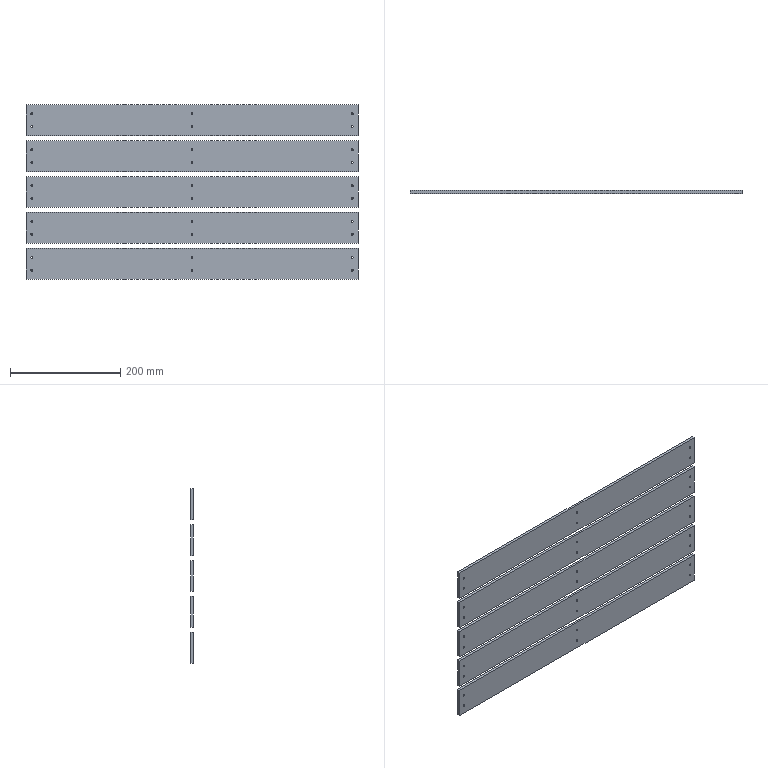CAM job | Mastercam | mm | 4 operations | part box 601 x 5 x 316
1. Contour (Ramp) | 3 - 3 平铣刀
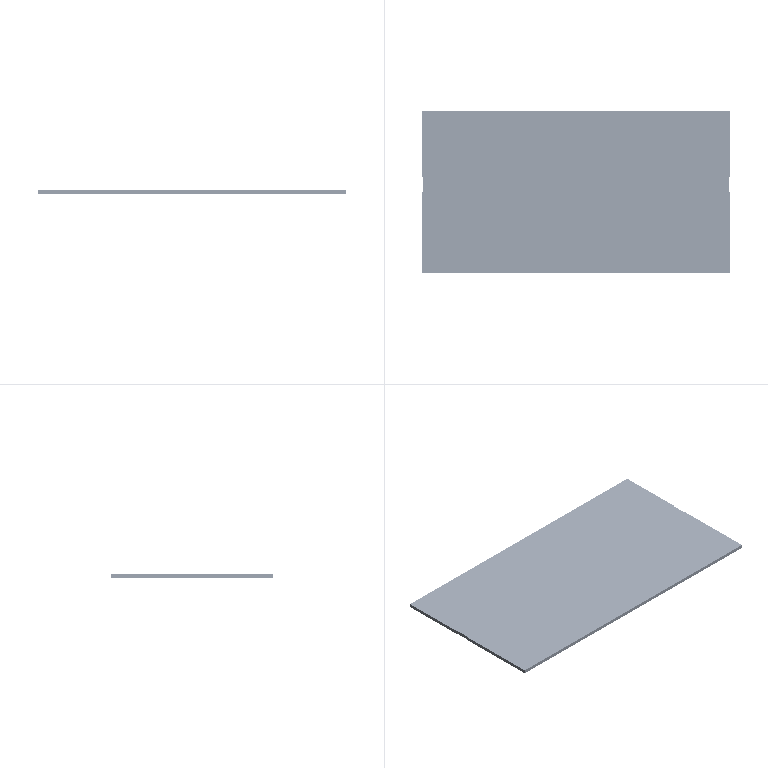2. Drill/Counterbore | 7 - 4 倒角刀
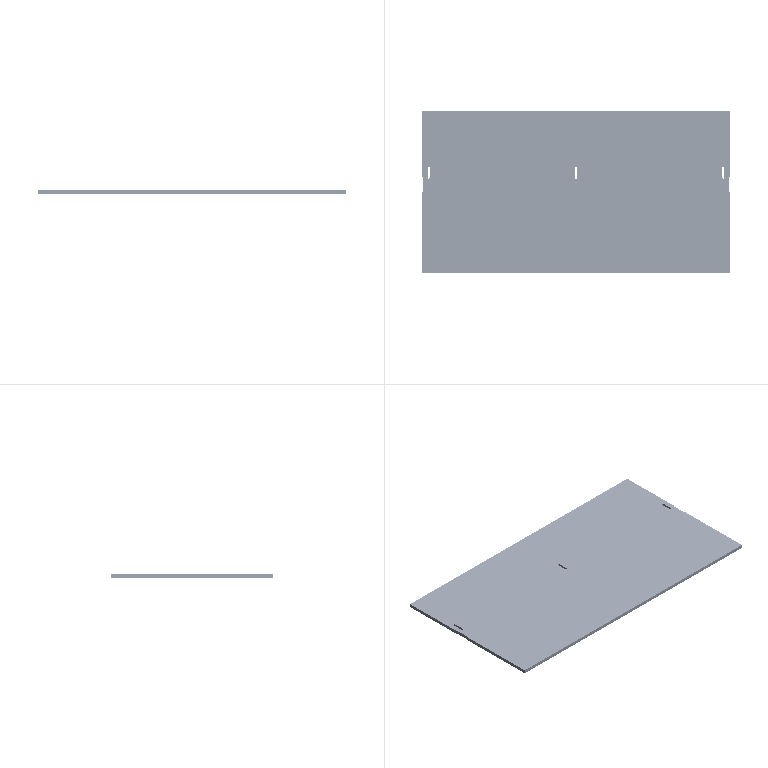3. Contour (2D chamfer) | 7 - 4 倒角刀
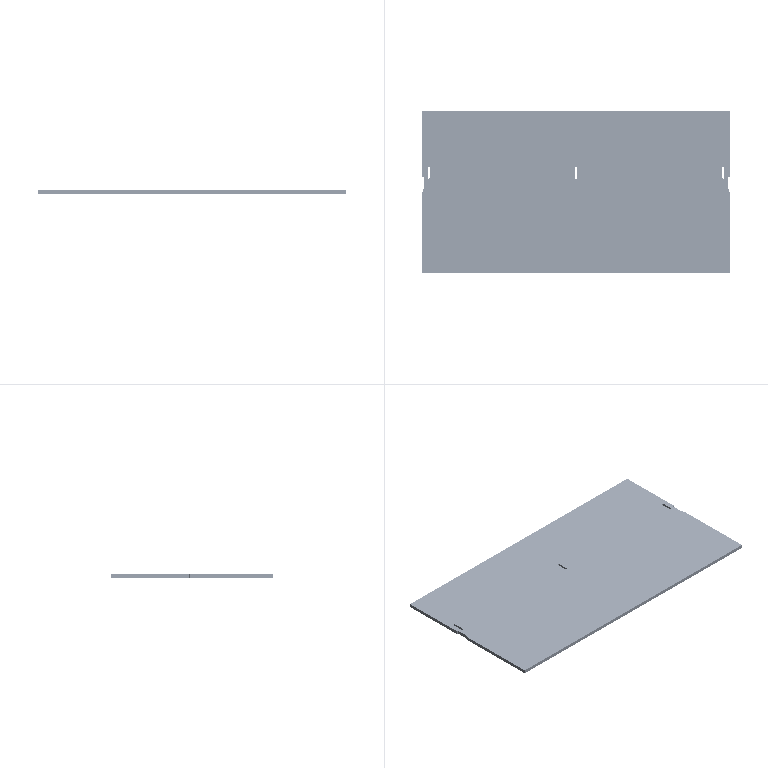4. Contour (Ramp) | 2 - 2 平铣刀